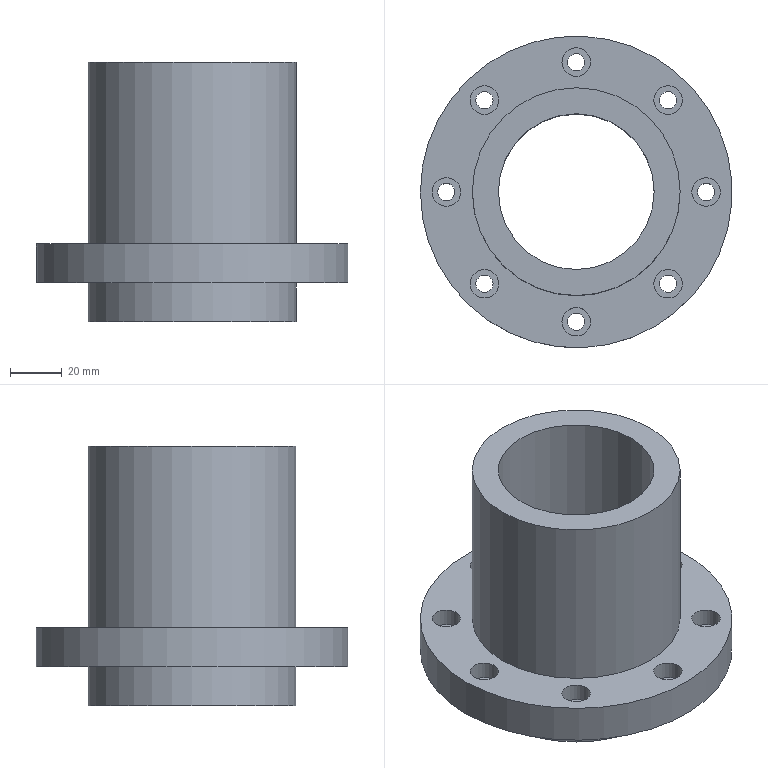Component | NX | LINEAR_BEARING | 1 solid | 32 faces | volume 306745 mm3 | cylinder 20 | plane 12 | commonest cylinder face diameters 6.6 x8 11 x8 80 x2 120 x1 60 x1